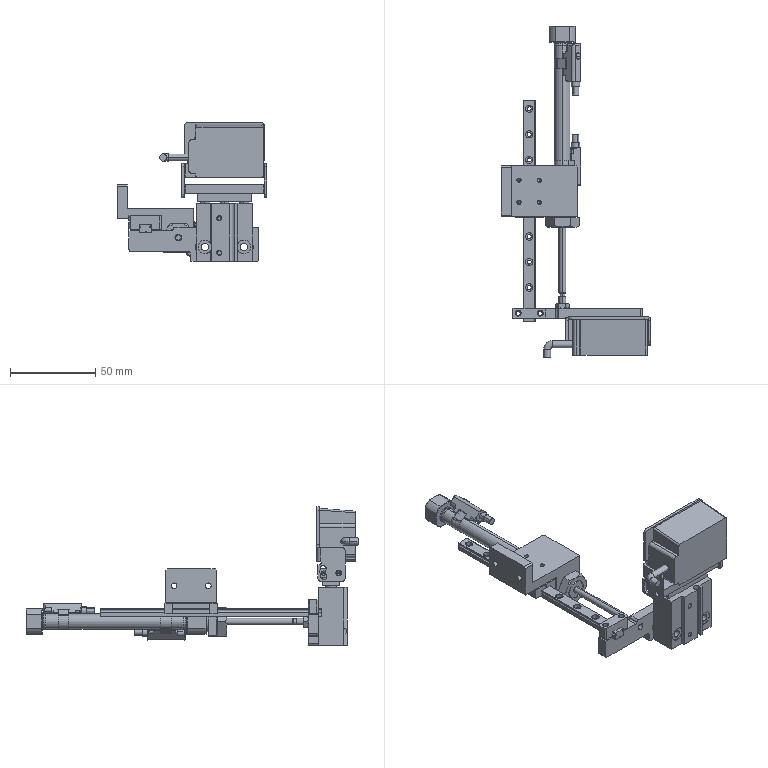Assembly | SolidWorks | mm | 16 component files | 16 solids | 812 faces | box 88 x 194.94 x 81.5 mm | volume 87527 mm3 | cylinder 341 | plane 325 | cone 110 | torus 30 | sphere 4 | spline 2 | commonest cylinder face diameters 2 x39 2.5 x28 0.6 x28 4 x22 2.4 x18 3.5 x17 3.4 x16 6 x12
Bill of materials:
BL-1300 | 1 |  | Rectangular box-shaped body with slightly rounded edges, a thin stepped flange/plate on one end face, and a small round rod that sticks out of that end and bends 90 degrees.
F01AE00111-A5175 | 1 | 6061 Alloy | Elongated rectangular block with chamfered corners in plan view, two vertical through-holes near the ends, and a rectangular notch cut across the underside, giving a bridge-like profile.
F01AE00111-A5207 | 1 |  | Flat rectangular bar with slightly chamfered corners, two through-holes in the main face near the center, and a smaller hole in each end face with a conical (drill-point) bottom.
F01AE00111-A5211 | 1 |  | Bracket with a horizontal plate, an upright flange along one edge, and a downward lug on the opposite side that has a large round bore. Several small holes are in the plate and flange.
F01AE00111-A5212 | 1 |  | Long flat bar/arm with a stepped outline. One end has a narrower section with a top notch and small holes; the wider section has one round through-hole and a long through-slot with rounded ends.
F01AE00111-A5219 | 1 |  | Sheet-metal-style U-shaped bracket: a rectangular back plate with two side tabs bent perpendicular. It has slots and holes, plus bend-relief cutouts.
MANIFOLD_SOLID_BREP_40_1 | 1 |  | Long, narrow straight bar with a profiled cross-section (groove along each side) and a row of evenly spaced counterbored-looking holes through the top along its length.
MANIFOLD_SOLID_BREP_81 | 1 |  | Rectangular block with a channel along its underside (inverted-U end profile), four holes in the top face, a groove line separating an end section, and small holes on the end face.
1-11 | 1 |  | Rectangular block with stepped and V-notched edges, two large and one smaller vertical through-hole, a partial-cylinder groove along one face, and cross holes on the sides.
2-11 | 1 |  | Rectangular plate with three parallel cylindrical posts hanging from its underside. The middle post ends in a larger disc/collar, and the plate has two small through-holes.
Mates:
1. concentric | F01AE00111-A5211-1 face at (-44.181, -50.188, -311.979) dir (0, -1, 0) r 6.25 | MI-8x60-S-U-M-2(0)-1/MI 8x60-S-U_c-1 face at (-44.181, -44.188, -311.979) dir (0, -1, 0) r 6
2. coincident | F01AE00111-A5212-1 face at (-12.181, -103.773, -316.979) dir (0, 1, 0) | MI-8x60-S-U-M-2(0)-1/MI8-M4x0_7 - Nut-2 face at (-44.181, -103.773, -311.979) dir (0, -1, 0)
3. parallel | F01AE00111-A5211-1 face at (-57.681, -35.188, -320.979) dir (0, 0, -1) | MI-8x60-S-U-M-2(0)-1/MI8-M12x1_25 - Nut-1 face at (-39.273, -44.188, -320.479) dir (0, 0, -1)
4. coincident | F01AE00111-A5211-1 face at (-80.181, -50.188, -294.979) dir (0, -1, 0) | MI-8x60-S-U-M-2(0)-1/MI8-M12x1_25 - Nut-1 face at (-36.181, -50.188, -311.979) dir (0, 1, 0)
5. coincident | F01AE00111-A5207-1 face at (-40.681, -124.273, -285.979) dir (0, 0, -1) | MGJ10-15-1/2-11-1 face at (-17.181, -117.273, -285.979) dir (0, 0, 1)
6. width | MGJ10-15-1/2-11-1 face at (-1.181, -122.273, -290.979) dir (0, -1, 0) | MGJ10-15-1/2-11-1 face at (-33.181, -112.273, -290.979) dir (0, 1, 0) | F01AE00111-A5207-1 face at (-40.681, -110.273, -285.979) dir (0, 1, 0) | F01AE00111-A5207-1 face at (-40.681, -124.273, -280.979) dir (0, -1, 0)
7. width | F01AE00111-A5207-1 face at (6.319, -124.273, -285.979) dir (1, 0, 0) | F01AE00111-A5207-1 face at (-40.681, -124.273, -285.979) dir (-1, 0, 0) | MGJ10-15-1/2-11-1 face at (-33.181, -122.273, -290.979) dir (-1, 0, 0) | MGJ10-15-1/2-11-1 face at (-1.181, -112.273, -290.979) dir (1, 0, 0)
8. coincident | F01AE00111-A5212-1 face at (-12.181, -109.773, -316.979) dir (0, -1, 0) | MGJ10-15-1/1-11-1 face at (-0.6807, -109.773, -291.979) dir (0, 1, 0)
9. coincident | F01AE00111-A5212-1 edge at (-36.181, -109.773, -325.979) dir (1, 0, 0) | MGJ10-15-1/1-11-1 face at (-17.181, -117.273, -325.979) dir (0, 0, -1)
10. width | F01AE00111-A5212-1 face at (-37.181, -103.773, -325.979) dir (-1, 0, 0) | F01AE00111-A5212-1 face at (2.819, -109.773, -325.979) dir (1, 0, 0) | MGJ10-15-1/1-11-1 face at (-0.6807, -126.773, -291.979) dir (1, 0, 0) | MGJ10-15-1/1-11-1 face at (-33.681, -109.773, -291.979) dir (-1, 0, 0)
11. concentric | F01AE00111-A5212-1 face at (-44.181, -103.773, -311.979) dir (0, 1, 0) r 2 | MI-8x60-S-U-M-2(0)-1/MI 8x60-S-U_r-1 face at (-44.181, 11.727, -311.979) dir (0, -1, 0) r 2
12. coincident | F01AE00111-A5212-1 face at (-67.181, -103.773, -308.979) dir (0, 0, 1) | MANIFOLD_SOLID_BREP_40_1-1 face at (-67.181, -21.773, -308.979) dir (0, 0, -1)
13. coincident | F01AE00111-A5211-1 face at (-57.681, -35.188, -300.979) dir (0, 0, -1) | MANIFOLD_SOLID_BREP_81-2 face at (-55.181, -19.788, -300.979) dir (0, 0, 1)
14. concentric | F01AE00111-A5211-1 face at (-57.681, -41.688, -320.979) dir (0, 0, 1) r 1.25 | MANIFOLD_SOLID_BREP_81-2 face at (-57.681, -41.688, -300.979) dir (0, 0, 1) r 1
15. concentric | F01AE00111-A5211-1 edge at (-69.681, -41.688, -294.979) dir (0, 0, 1) r 1.25 | MANIFOLD_SOLID_BREP_81-2 face at (-69.681, -41.688, -300.979) dir (0, 0, 1) r 1
16. concentric | MANIFOLD_SOLID_BREP_81-2 face at (-67.181, -15.188, -305.679) dir (0, -1, 0) r 0.7 | MANIFOLD_SOLID_BREP_40_1-1 face at (-67.181, -21.773, -305.679) dir (0, 1, 0) r 0.7
17. concentric | F01AE00111-A5212-1 face at (-63.681, -106.773, -308.979) dir (0, 0, 1) r 0.8 | MANIFOLD_SOLID_BREP_40_1-1 face at (-63.681, -106.773, -304.179) dir (0, 0, 1) r 1.2
18. coincident | MANIFOLD_SOLID_BREP_40_1-1 face at (-60.181, -21.773, -304.179) dir (0, 0, 1) | F01AE00111-A5175-1 face at (-60.181, -103.773, -304.179) dir (0, 0, -1)
19. width | F01AE00111-A5175-1 face at (-63.681, -109.773, -304.179) dir (0, -1, 0) | F01AE00111-A5175-1 face at (-63.681, -103.773, -304.179) dir (0, 1, 0) | F01AE00111-A5212-1 face at (-12.181, -109.773, -316.979) dir (0, -1, 0) | F01AE00111-A5212-1 face at (-12.181, -103.773, -316.979) dir (0, 1, 0)
20. width | F01AE00111-A5175-1 face at (-60.181, -103.773, -304.179) dir (-1, 0, 0) | F01AE00111-A5175-1 face at (-67.181, -103.773, -304.179) dir (1, 0, 0) | MANIFOLD_SOLID_BREP_40_1-1 face at (-60.181, -21.773, -308.979) dir (1, 0, 0) | MANIFOLD_SOLID_BREP_40_1-1 face at (-67.181, -21.773, -306.379) dir (-1, 0, 0)
21. coincident | BL-1300-2 face at (5.719, -110.523, -276.479) dir (0, 1, 0) | F01AE00111-A5219-1 face at (22.319, -110.523, -288.479) dir (0, -1, 0)
22. parallel | F01AE00111-A5207-1 face at (-40.681, -124.273, -285.979) dir (0, 0, -1) | F01AE00111-A5219-1 face at (-42.181, -46.56, -288.479) dir (0, 0, -1)
23. concentric | BL-1300-2 face at (2.219, -110.523, -272.979) dir (0, 1, 0) r 1.25 | F01AE00111-A5219-1 face at (2.219, -109.023, -272.979) dir (0, -1, 0) r 1.75
24. parallel | F01AE00111-A5207-1 face at (-40.681, -124.273, -285.979) dir (0, 0, -1) | BL-1300-2 face at (5.719, -131.523, -276.479) dir (0, 0, -1)
25. width | F01AE00111-A5219-1 face at (6.319, -125.56, -288.479) dir (-1, 0, 0) | F01AE00111-A5219-1 face at (-40.681, -46.56, -288.479) dir (1, 0, 0) | F01AE00111-A5207-1 face at (6.319, -124.273, -285.979) dir (1, 0, 0) | F01AE00111-A5207-1 face at (-40.681, -124.273, -285.979) dir (-1, 0, 0)
26. concentric | F01AE00111-A5207-1 face at (6.319, -121.773, -283.479) dir (1, 0, 0) r 1.25 | F01AE00111-A5219-1 face at (-42.184, -121.773, -283.479) dir (1, 0, 0) r 1.75
27. coincident | MI 8x60-S-U_c-1 axis at (-80.9, 0, 0) dir (1, 0, 0) | MI 8x60-S-U_r-1 axis at (82.775, 0, 0) dir (-1, 0, 0)
28. angle | MI 8x60-S-U_r-1 plane at (1.875, 0, 0) dir (0, 0, -1) | MI 8x60-S-U_c-1 plane at (0, 0, 0) dir (0, 0, -1)
29. coincident | MI 8x60-S-U_r-1 axis at (-79.025, 0, 0) dir (1, 0, 0) | MI8-M4x0_7 - Nut-2 axis at (58.275, 0, 0) dir (-1, 0, 0)
30. angle | MI8-M4x0_7 - Nut-2 plane at (-22.625, 0, 0) dir (0, 0, -1) | MI 8x60-S-U_r-1 plane at (1.875, 0, 0) dir (0, 0, -1)
31. coincident | MI 8x60-S-U_c-1 axis at (-80.9, 0, 0) dir (1, 0, 0) | MI8-M12x1_25 - Nut-1 axis at (68.9, 0, 0) dir (-1, 0, 0)
32. angle | MI8-M12x1_25 - Nut-1 plane at (-12, 0, 0) dir (0, 0, -1) | MI 8x60-S-U_c-1 plane at (0, 0, 0) dir (0, 0, -1)
33. distance | CS1-M-S8-1 plane at (12.5, 0, 0) dir (1, 0, 0) | MI 8x60-S-U_c-1 plane at (12.5, 0, 0) dir (-1, 0, 0)
34. coincident | MI 8x60-S-U_c-1 axis at (-80.9, 0, 0) dir (1, 0, 0) | CS1-M-S8-1 axis at (93.4, 0, 0) dir (-1, 0, 0)
35. angle | CS1-M-S8-1 plane at (12.5, 0, 0) dir (0, 0.7071, -0.7071) | MI 8x60-S-U_c-1 plane at (0, 0, 0) dir (0, 0, -1)
36. distance | CS1-M-S8-2 plane at (95.5, 0, 0) dir (-1, 0, 0) | MI 8x60-S-U_c-1 plane at (95.5, 0, 0) dir (1, 0, 0)
37. coincident | MI 8x60-S-U_c-1 axis at (80.9, 0, 0) dir (-1, 0, 0) | CS1-M-S8-2 axis at (14.6, 0, 0) dir (1, 0, 0)
38. angle | CS1-M-S8-2 plane at (95.5, 0, 0) dir (0, 0.7071, 0.7071) | MI 8x60-S-U_c-1 plane at (0, 0, 0) dir (0, 0, -1)
39. distance | MI8-M4x0_7 - Nut-2 face at (-22.625, 0, 0) dir (-1, 0, 0) | MI 8x60-S-U_r-1 face at (-26.125, 0, 0) dir (-1, 0, 0)
40. concentric | MI 8x60-S-U_c-1 face at (91, 0, 0) dir (-1, 0, 0) r 2 | MI 8x60-S-U_r-1 face at (92.875, 0, 0) dir (-1, 0, 0) r 2
41. distance | MI 8x60-S-U_r-1 face at (-26.125, 0, 0) dir (-1, 0, 0) | MI 8x60-S-U_c-1 face at (-12, 0, 0) dir (-1, 0, 0)
42. coincident | MI 8x60-S-U_c-1 face at (-12, 0, 0) dir (-1, 0, 0) | MI8-M12x1_25 - Nut-1 face at (-12, 0, 0) dir (-1, 0, 0)